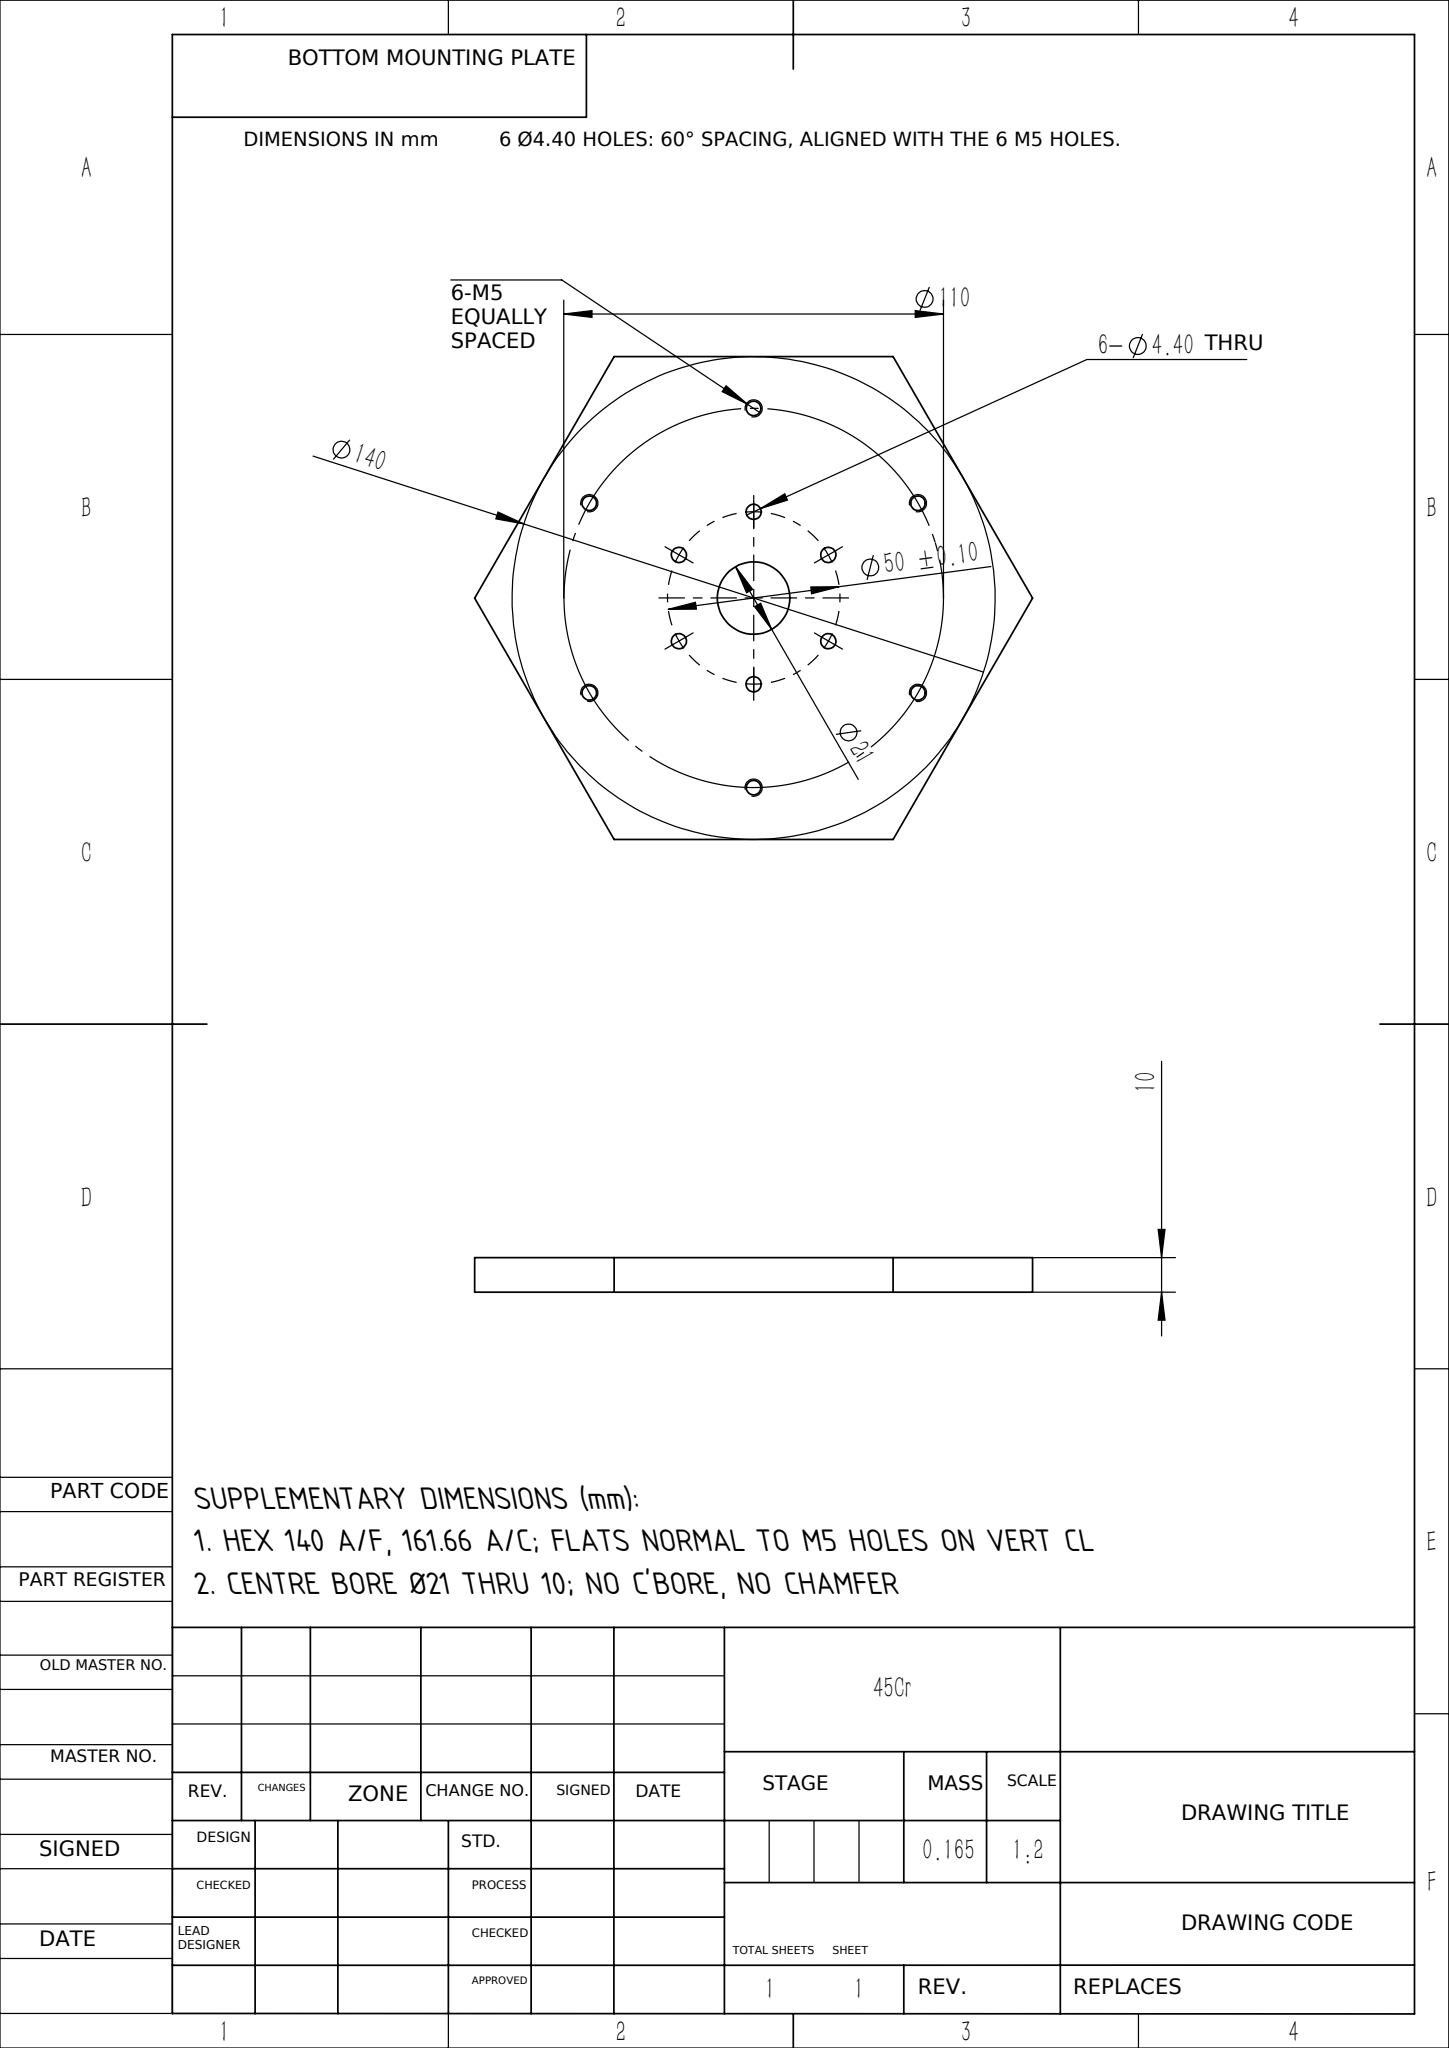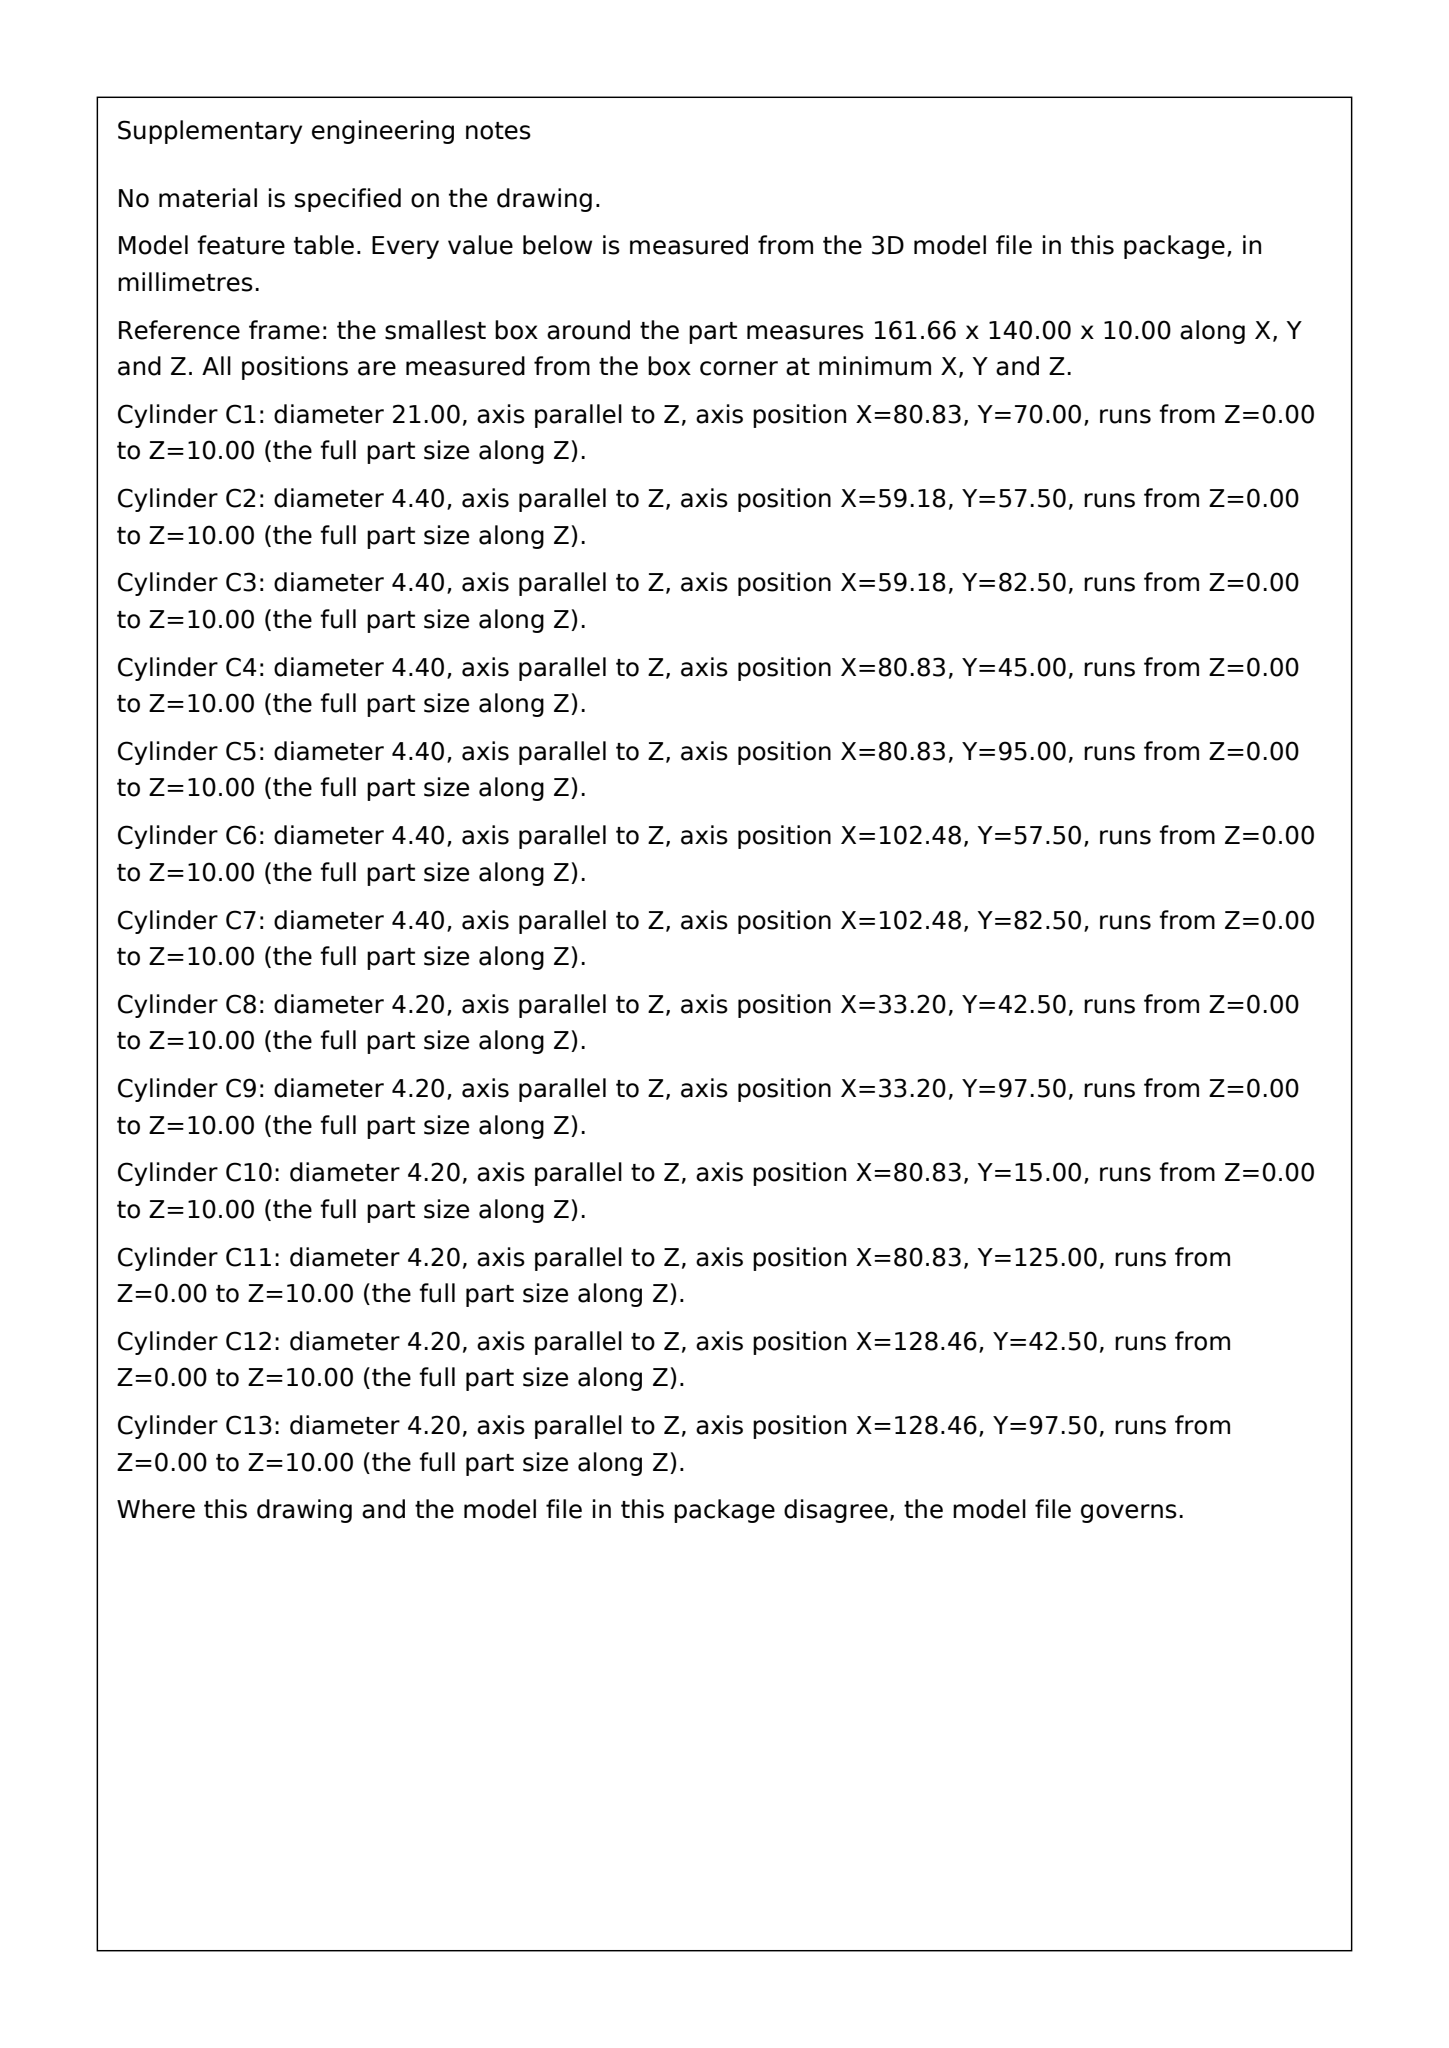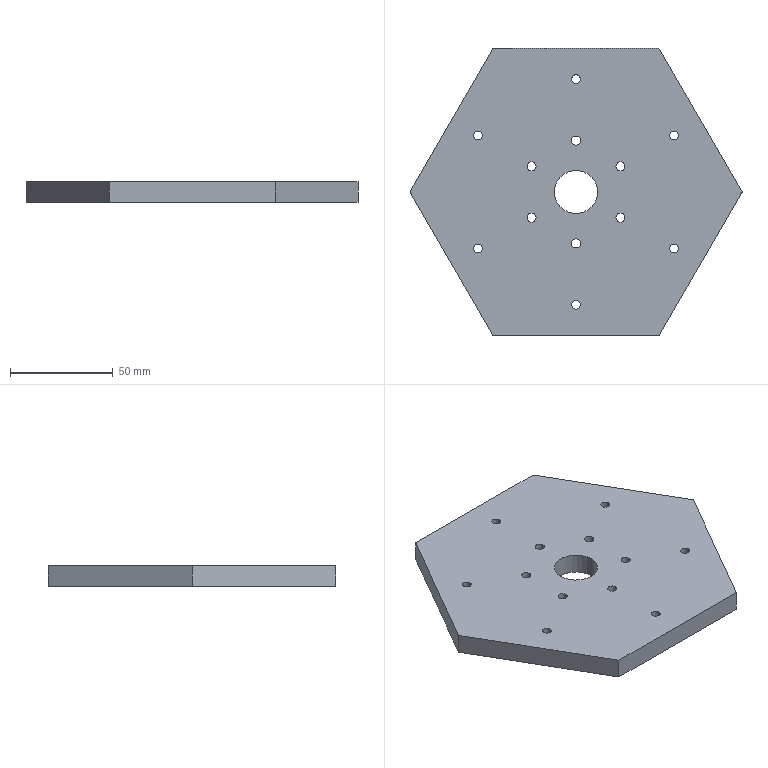Part | SolidWorks | mm | 1 solid | 34 faces | box 161.66 x 140 x 10 mm | volume 164534 mm3 | cylinder 26 | plane 8 | commonest cylinder face diameters 4.2 x12 4.4 x12 21 x2
build123d program:
from build123d import *

# Parameters (mm, degrees)
BOSS_EXTRUDE1_DEPTH = 5
SKETCH2_R           = 10.5
CUT_EXTRUDE1_DEPTH  = 10
SKETCH3_R           = 2.2
CUT_EXTRUDE2_DEPTH  = 10
CIRPATTERN1_COUNT   = 6
SKETCH4_R           = 1.5
CUT_EXTRUDE3_DEPTH  = 10
CIRPATTERN2_COUNT   = 6


with BuildPart() as part:
    # Sketch1 → Boss-Extrude1 (new, symmetric)
    with BuildSketch(Plane.XY):
        Polygon((-40.415, 70), (-80.829, 0), (-40.415, -70), (40.415, -70), (80.829, 0), (40.415, 70), align=None)
    extrude(amount=BOSS_EXTRUDE1_DEPTH, both=True)

    # Sketch2 → Cut-Extrude1 (cut)
    with BuildSketch(Plane.XY.offset(5)):
        Circle(SKETCH2_R)
    extrude(amount=-CUT_EXTRUDE1_DEPTH, mode=Mode.SUBTRACT)

    # Sketch3 → Cut-Extrude2 (cut)
    with BuildSketch(Plane(origin=(0, 0, -5), x_dir=(-1, 0, 0), z_dir=(0, 0, -1))):
        with Locations((0, 25)):
            Circle(SKETCH3_R)
    cut_extrude2 = extrude(amount=-CUT_EXTRUDE2_DEPTH, mode=Mode.SUBTRACT)

    # CirPattern1: Cut-Extrude2 ×6 about axis
    cirpattern1_axis = Axis((0, 0, 0), (0, 0, 1))
    for i in range(1, CIRPATTERN1_COUNT):
        add(cut_extrude2.rotate(cirpattern1_axis, i * 360 / CIRPATTERN1_COUNT), mode=Mode.SUBTRACT)

    # Sketch4 → Cut-Extrude3 (cut)
    with BuildSketch(Plane(origin=(0, 0, -5), x_dir=(-1, 0, 0), z_dir=(0, 0, -1))):
        with Locations((0, 55)):
            Circle(SKETCH4_R)
    cut_extrude3 = extrude(amount=-CUT_EXTRUDE3_DEPTH, mode=Mode.SUBTRACT)

    # Sketch6 → M5x0.8 Tapped Hole1 (revolve, cut)
    with BuildSketch(Plane(origin=(0, 55, -5), x_dir=(0, 1, 0), z_dir=(1, 0, 0))):
        Polygon((0, 0), (0, 13.662), (2.1, 12.4), (2.1, 0), align=None)
    m5x0_8_tapped_hole1 = revolve(axis=Axis((0, 55, -11.35), (0, 0, 1)), mode=Mode.SUBTRACT)

    # CirPattern2: Cut-Extrude3, M5x0.8 Tapped Hole1 ×6 about axis
    cirpattern2_axis = Axis((0, 0, 0), (0, 0, 1))
    add([cut_extrude3.rotate(cirpattern2_axis, i * 360 / CIRPATTERN2_COUNT) for i in range(1, CIRPATTERN2_COUNT)], mode=Mode.SUBTRACT)
    add([m5x0_8_tapped_hole1.rotate(cirpattern2_axis, i * 360 / CIRPATTERN2_COUNT) for i in range(1, CIRPATTERN2_COUNT)], mode=Mode.SUBTRACT)


solid = part.part